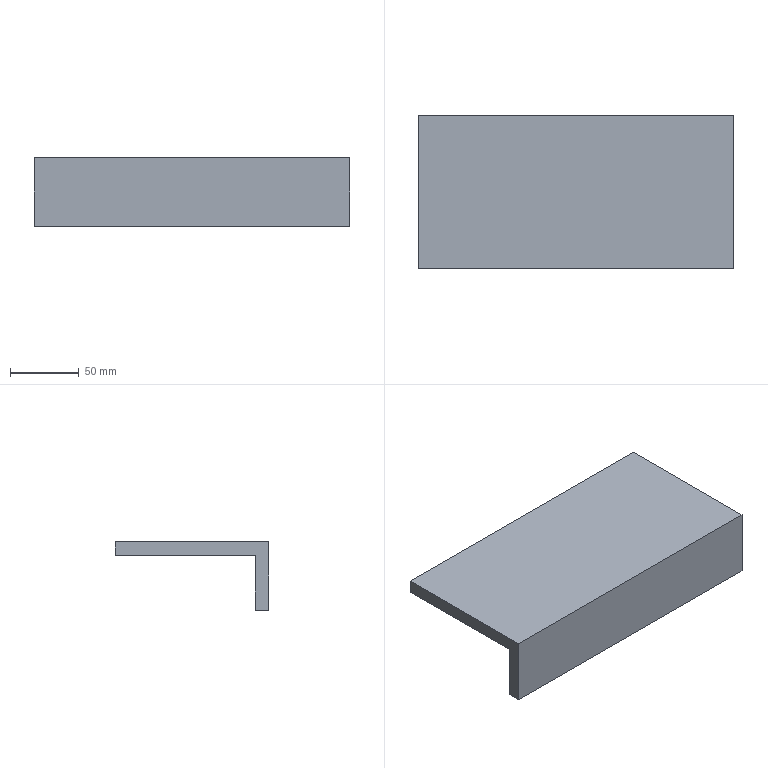Component | SolidWorks | BearingLiftingModule-1_CHEN123-AA-21-1 | 1 solid | 8 faces | box 230 x 112 x 50 mm | volume 349600 mm3 | plane 8
build123d program:
from build123d import *

# Parameters (mm, degrees)
BOSS_EXTRUDE1_DEPTH = 115


with BuildPart() as part:
    # Sketch1 → Boss-Extrude1 (new, symmetric)
    with BuildSketch(Plane.XY):
        Polygon((0, 0), (0, 112), (-10, 112), (-10, 10), (-50, 10), (-50, 0), align=None)
    extrude(amount=BOSS_EXTRUDE1_DEPTH, both=True)


solid = part.part

# Placed as in the assembly
solid = solid.moved(Location((34.999, -150.999, 10), (0, -90, 0)))
STEP:
#1=COLOUR_RGB('',0.7922,0.8196,0.9333);
#2=FILL_AREA_STYLE_COLOUR('',#1);
#3=FILL_AREA_STYLE('',(#2));
#4=SURFACE_STYLE_FILL_AREA(#3);
#5=SURFACE_SIDE_STYLE('',(#4));
#6=SURFACE_STYLE_USAGE(.BOTH.,#5);
#7=PRESENTATION_STYLE_ASSIGNMENT((#6));
#8=CARTESIAN_POINT('',(5.905,-5.945,-1.575));
#9=VERTEX_POINT('',#8);
#10=CARTESIAN_POINT('',(5.905,-5.945,0.3937));
#11=VERTEX_POINT('',#10);
#12=CARTESIAN_POINT('',(5.905,-5.945,0.3937));
#13=DIRECTION('',(0.,0.,1.));
#14=VECTOR('',#13,39.37);
#15=LINE('',#12,#14);
#16=EDGE_CURVE('',#9,#11,#15,.T.);
#17=ORIENTED_EDGE('',*,*,#16,.T.);
#18=CARTESIAN_POINT('',(-3.15,-5.945,0.3937));
#19=VERTEX_POINT('',#18);
#20=CARTESIAN_POINT('',(-3.15,-5.945,0.3937));
#21=DIRECTION('',(1.,0.,0.));
#22=VECTOR('',#21,39.37);
#23=LINE('',#20,#22);
#24=EDGE_CURVE('',#19,#11,#23,.T.);
#25=ORIENTED_EDGE('',*,*,#24,.F.);
#26=CARTESIAN_POINT('',(-3.15,-5.945,-1.575));
#27=VERTEX_POINT('',#26);
#28=CARTESIAN_POINT('',(-3.15,-5.945,0.3937));
#29=DIRECTION('',(0.,0.,1.));
#30=VECTOR('',#29,39.37);
#31=LINE('',#28,#30);
#32=EDGE_CURVE('',#27,#19,#31,.T.);
#33=ORIENTED_EDGE('',*,*,#32,.F.);
#34=CARTESIAN_POINT('',(-3.15,-5.945,-1.575));
#35=DIRECTION('',(1.,0.,0.));
#36=VECTOR('',#35,39.37);
#37=LINE('',#34,#36);
#38=EDGE_CURVE('',#27,#9,#37,.T.);
#39=ORIENTED_EDGE('',*,*,#38,.T.);
#40=EDGE_LOOP('',(#17,#25,#33,#39));
#41=FACE_OUTER_BOUND('',#40,.T.);
#42=CARTESIAN_POINT('',(-3.15,-5.945,0.3937));
#43=DIRECTION('',(0.,1.,0.));
#44=DIRECTION('',(-1.,0.,0.));
#45=AXIS2_PLACEMENT_3D('',#42,#43,#44);
#46=PLANE('',#45);
#47=ADVANCED_FACE('',(#41),#46,.F.);
#48=CARTESIAN_POINT('',(5.905,-1.535,0.3937));
#49=VERTEX_POINT('',#48);
#50=CARTESIAN_POINT('',(5.905,-5.945,0.3937));
#51=DIRECTION('',(0.,1.,0.));
#52=VECTOR('',#51,39.37);
#53=LINE('',#50,#52);
#54=EDGE_CURVE('',#11,#49,#53,.T.);
#55=ORIENTED_EDGE('',*,*,#54,.T.);
#56=CARTESIAN_POINT('',(-3.15,-1.535,0.3937));
#57=VERTEX_POINT('',#56);
#58=CARTESIAN_POINT('',(-3.15,-1.535,0.3937));
#59=DIRECTION('',(1.,0.,0.));
#60=VECTOR('',#59,39.37);
#61=LINE('',#58,#60);
#62=EDGE_CURVE('',#57,#49,#61,.T.);
#63=ORIENTED_EDGE('',*,*,#62,.F.);
#64=CARTESIAN_POINT('',(-3.15,-5.945,0.3937));
#65=DIRECTION('',(0.,1.,0.));
#66=VECTOR('',#65,39.37);
#67=LINE('',#64,#66);
#68=EDGE_CURVE('',#19,#57,#67,.T.);
#69=ORIENTED_EDGE('',*,*,#68,.F.);
#70=ORIENTED_EDGE('',*,*,#24,.T.);
#71=EDGE_LOOP('',(#55,#63,#69,#70));
#72=FACE_OUTER_BOUND('',#71,.T.);
#73=CARTESIAN_POINT('',(-3.15,-5.945,0.3937));
#74=DIRECTION('',(0.,0.,-1.));
#75=DIRECTION('',(-1.,0.,0.));
#76=AXIS2_PLACEMENT_3D('',#73,#74,#75);
#77=PLANE('',#76);
#78=ADVANCED_FACE('',(#72),#77,.F.);
#79=CARTESIAN_POINT('',(5.905,-1.535,-0.));
#80=VERTEX_POINT('',#79);
#81=CARTESIAN_POINT('',(5.905,-1.535,-0.));
#82=DIRECTION('',(0.,0.,-1.));
#83=VECTOR('',#82,39.37);
#84=LINE('',#81,#83);
#85=EDGE_CURVE('',#49,#80,#84,.T.);
#86=ORIENTED_EDGE('',*,*,#85,.T.);
#87=CARTESIAN_POINT('',(-3.15,-1.535,-0.));
#88=VERTEX_POINT('',#87);
#89=CARTESIAN_POINT('',(-3.15,-1.535,-0.));
#90=DIRECTION('',(1.,0.,0.));
#91=VECTOR('',#90,39.37);
#92=LINE('',#89,#91);
#93=EDGE_CURVE('',#88,#80,#92,.T.);
#94=ORIENTED_EDGE('',*,*,#93,.F.);
#95=CARTESIAN_POINT('',(-3.15,-1.535,-0.));
#96=DIRECTION('',(0.,0.,-1.));
#97=VECTOR('',#96,39.37);
#98=LINE('',#95,#97);
#99=EDGE_CURVE('',#57,#88,#98,.T.);
#100=ORIENTED_EDGE('',*,*,#99,.F.);
#101=ORIENTED_EDGE('',*,*,#62,.T.);
#102=EDGE_LOOP('',(#86,#94,#100,#101));
#103=FACE_OUTER_BOUND('',#102,.T.);
#104=CARTESIAN_POINT('',(-3.15,-1.535,-0.));
#105=DIRECTION('',(0.,-1.,0.));
#106=DIRECTION('',(1.,0.,0.));
#107=AXIS2_PLACEMENT_3D('',#104,#105,#106);
#108=PLANE('',#107);
#109=ADVANCED_FACE('',(#103),#108,.F.);
#110=CARTESIAN_POINT('',(5.905,-5.551,-0.));
#111=VERTEX_POINT('',#110);
#112=CARTESIAN_POINT('',(5.905,-5.551,-0.));
#113=DIRECTION('',(0.,-1.,-0.));
#114=VECTOR('',#113,39.37);
#115=LINE('',#112,#114);
#116=EDGE_CURVE('',#80,#111,#115,.T.);
#117=ORIENTED_EDGE('',*,*,#116,.T.);
#118=CARTESIAN_POINT('',(-3.15,-5.551,-0.));
#119=VERTEX_POINT('',#118);
#120=CARTESIAN_POINT('',(-3.15,-5.551,-0.));
#121=DIRECTION('',(1.,0.,0.));
#122=VECTOR('',#121,39.37);
#123=LINE('',#120,#122);
#124=EDGE_CURVE('',#119,#111,#123,.T.);
#125=ORIENTED_EDGE('',*,*,#124,.F.);
#126=CARTESIAN_POINT('',(-3.15,-5.551,-0.));
#127=DIRECTION('',(0.,-1.,-0.));
#128=VECTOR('',#127,39.37);
#129=LINE('',#126,#128);
#130=EDGE_CURVE('',#88,#119,#129,.T.);
#131=ORIENTED_EDGE('',*,*,#130,.F.);
#132=ORIENTED_EDGE('',*,*,#93,.T.);
#133=EDGE_LOOP('',(#117,#125,#131,#132));
#134=FACE_OUTER_BOUND('',#133,.T.);
#135=CARTESIAN_POINT('',(-3.15,-5.551,-0.));
#136=DIRECTION('',(0.,-0.,1.));
#137=DIRECTION('',(0.,1.,0.));
#138=AXIS2_PLACEMENT_3D('',#135,#136,#137);
#139=PLANE('',#138);
#140=ADVANCED_FACE('',(#134),#139,.F.);
#141=CARTESIAN_POINT('',(5.905,-5.551,-1.575));
#142=VERTEX_POINT('',#141);
#143=CARTESIAN_POINT('',(5.905,-5.551,-1.575));
#144=DIRECTION('',(0.,0.,-1.));
#145=VECTOR('',#144,39.37);
#146=LINE('',#143,#145);
#147=EDGE_CURVE('',#111,#142,#146,.T.);
#148=ORIENTED_EDGE('',*,*,#147,.T.);
#149=CARTESIAN_POINT('',(-3.15,-5.551,-1.575));
#150=VERTEX_POINT('',#149);
#151=CARTESIAN_POINT('',(-3.15,-5.551,-1.575));
#152=DIRECTION('',(1.,0.,0.));
#153=VECTOR('',#152,39.37);
#154=LINE('',#151,#153);
#155=EDGE_CURVE('',#150,#142,#154,.T.);
#156=ORIENTED_EDGE('',*,*,#155,.F.);
#157=CARTESIAN_POINT('',(-3.15,-5.551,-1.575));
#158=DIRECTION('',(0.,0.,-1.));
#159=VECTOR('',#158,39.37);
#160=LINE('',#157,#159);
#161=EDGE_CURVE('',#119,#150,#160,.T.);
#162=ORIENTED_EDGE('',*,*,#161,.F.);
#163=ORIENTED_EDGE('',*,*,#124,.T.);
#164=EDGE_LOOP('',(#148,#156,#162,#163));
#165=FACE_OUTER_BOUND('',#164,.T.);
#166=CARTESIAN_POINT('',(-3.15,-5.551,-1.575));
#167=DIRECTION('',(0.,-1.,0.));
#168=DIRECTION('',(1.,0.,0.));
#169=AXIS2_PLACEMENT_3D('',#166,#167,#168);
#170=PLANE('',#169);
#171=ADVANCED_FACE('',(#165),#170,.F.);
#172=CARTESIAN_POINT('',(5.905,-5.945,-1.575));
#173=DIRECTION('',(0.,-1.,0.));
#174=VECTOR('',#173,39.37);
#175=LINE('',#172,#174);
#176=EDGE_CURVE('',#142,#9,#175,.T.);
#177=ORIENTED_EDGE('',*,*,#176,.T.);
#178=ORIENTED_EDGE('',*,*,#38,.F.);
#179=CARTESIAN_POINT('',(-3.15,-5.945,-1.575));
#180=DIRECTION('',(0.,-1.,0.));
#181=VECTOR('',#180,39.37);
#182=LINE('',#179,#181);
#183=EDGE_CURVE('',#150,#27,#182,.T.);
#184=ORIENTED_EDGE('',*,*,#183,.F.);
#185=ORIENTED_EDGE('',*,*,#155,.T.);
#186=EDGE_LOOP('',(#177,#178,#184,#185));
#187=FACE_OUTER_BOUND('',#186,.T.);
#188=CARTESIAN_POINT('',(-3.15,-5.945,-1.575));
#189=DIRECTION('',(0.,0.,1.));
#190=DIRECTION('',(1.,0.,0.));
#191=AXIS2_PLACEMENT_3D('',#188,#189,#190);
#192=PLANE('',#191);
#193=ADVANCED_FACE('',(#187),#192,.F.);
#194=ORIENTED_EDGE('',*,*,#32,.T.);
#195=ORIENTED_EDGE('',*,*,#68,.T.);
#196=ORIENTED_EDGE('',*,*,#99,.T.);
#197=ORIENTED_EDGE('',*,*,#130,.T.);
#198=ORIENTED_EDGE('',*,*,#161,.T.);
#199=ORIENTED_EDGE('',*,*,#183,.T.);
#200=EDGE_LOOP('',(#194,#195,#196,#197,#198,#199));
#201=FACE_OUTER_BOUND('',#200,.T.);
#202=CARTESIAN_POINT('',(-3.15,-5.945,0.3937));
#203=DIRECTION('',(1.,0.,0.));
#204=DIRECTION('',(0.,0.,-1.));
#205=AXIS2_PLACEMENT_3D('',#202,#203,#204);
#206=PLANE('',#205);
#207=ADVANCED_FACE('',(#201),#206,.F.);
#208=ORIENTED_EDGE('',*,*,#16,.F.);
#209=ORIENTED_EDGE('',*,*,#176,.F.);
#210=ORIENTED_EDGE('',*,*,#147,.F.);
#211=ORIENTED_EDGE('',*,*,#116,.F.);
#212=ORIENTED_EDGE('',*,*,#85,.F.);
#213=ORIENTED_EDGE('',*,*,#54,.F.);
#214=EDGE_LOOP('',(#208,#209,#210,#211,#212,#213));
#215=FACE_OUTER_BOUND('',#214,.T.);
#216=CARTESIAN_POINT('',(5.905,-5.945,0.3937));
#217=DIRECTION('',(1.,0.,0.));
#218=DIRECTION('',(0.,0.,-1.));
#219=AXIS2_PLACEMENT_3D('',#216,#217,#218);
#220=PLANE('',#219);
#221=ADVANCED_FACE('',(#215),#220,.T.);
#222=CLOSED_SHELL('',(#47,#78,#109,#140,#171,#193,#207,#221));
#223=MANIFOLD_SOLID_BREP('',#222);
#224=STYLED_ITEM('',(#7),#223);
#225=(LENGTH_UNIT()NAMED_UNIT(*)SI_UNIT($,.METRE.));
#226=LENGTH_MEASURE_WITH_UNIT(LENGTH_MEASURE(0.0254),#225);
#227=DIMENSIONAL_EXPONENTS(1.,0.,0.,0.,0.,0.,0.);
#228=(CONVERSION_BASED_UNIT('',#226)LENGTH_UNIT()NAMED_UNIT(#227));
#229=UNCERTAINTY_MEASURE_WITH_UNIT(LENGTH_MEASURE(0.00001),#228,'','');
#230=(NAMED_UNIT(*)PLANE_ANGLE_UNIT()SI_UNIT($,.RADIAN.));
#231=(NAMED_UNIT(*)SI_UNIT($,.STERADIAN.)SOLID_ANGLE_UNIT());
#232=(GEOMETRIC_REPRESENTATION_CONTEXT(3)GLOBAL_UNCERTAINTY_ASSIGNED_CONTEXT((#229))GLOBAL_UNIT_ASSIGNED_CONTEXT((#228,#230,#231))REPRESENTATION_CONTEXT('',''));
#233=MECHANICAL_DESIGN_GEOMETRIC_PRESENTATION_REPRESENTATION('',(#224),#232);
#234=PRESENTATION_LAYER_ASSIGNMENT('','',(#224));
#235=CARTESIAN_POINT('',(0.,0.,0.));
#236=DIRECTION('',(0.,0.,1.));
#237=DIRECTION('',(1.,0.,0.));
#238=AXIS2_PLACEMENT_3D('',#235,#236,#237);
#239=(LENGTH_UNIT()NAMED_UNIT(*)SI_UNIT($,.METRE.));
#240=LENGTH_MEASURE_WITH_UNIT(LENGTH_MEASURE(0.0254),#239);
#241=DIMENSIONAL_EXPONENTS(1.,0.,0.,0.,0.,0.,0.);
#242=(CONVERSION_BASED_UNIT('',#240)LENGTH_UNIT()NAMED_UNIT(#241));
#243=UNCERTAINTY_MEASURE_WITH_UNIT(LENGTH_MEASURE(0.00001),#242,'','');
#244=(NAMED_UNIT(*)PLANE_ANGLE_UNIT()SI_UNIT($,.RADIAN.));
#245=(NAMED_UNIT(*)SI_UNIT($,.STERADIAN.)SOLID_ANGLE_UNIT());
#246=(GEOMETRIC_REPRESENTATION_CONTEXT(3)GLOBAL_UNCERTAINTY_ASSIGNED_CONTEXT((#243))GLOBAL_UNIT_ASSIGNED_CONTEXT((#242,#244,#245))REPRESENTATION_CONTEXT('',''));
#247=ADVANCED_BREP_SHAPE_REPRESENTATION('',(#223,#238),#246);